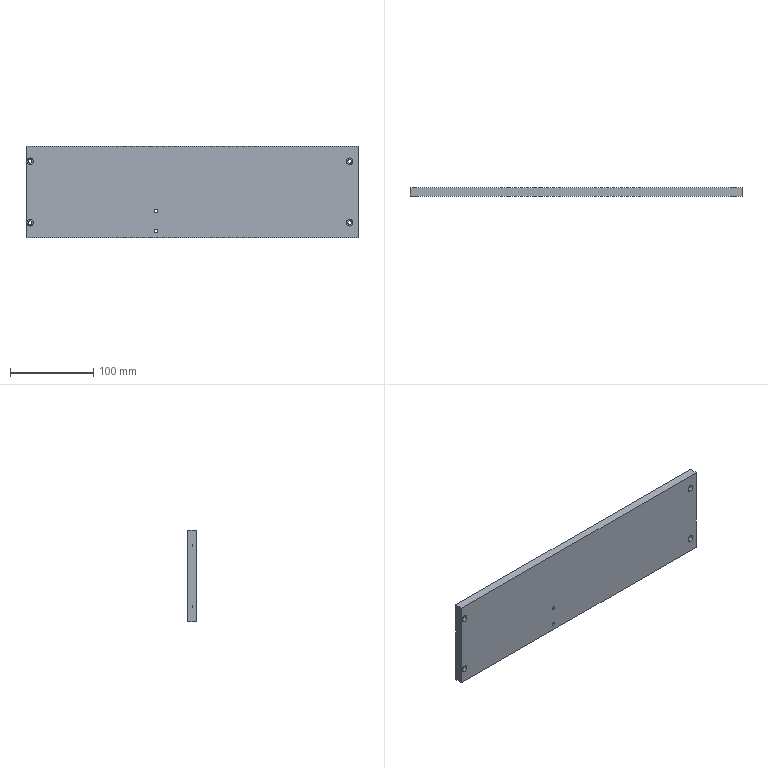Component | SolidWorks | CS021-A10-A001-1 | 1 solid | 30 faces | box 400 x 10 x 110 mm | volume 438454 mm3 | cylinder 20 | plane 10 | commonest cylinder face diameters 8 x8 4.5 x8 4.2 x4 | material AL6061
build123d program:
from build123d import *

# Parameters (mm, degrees)
SKETCH1_W                                          = 400
SKETCH1_H                                          = 110
BOSS_EXTRUDE1_DEPTH                                = 5
M5_TAPPED_HOLE1_D                                  = 4.2
HOLE_SIZE_ACCORDING_TO_SLOTTED_PAN_HEA_D           = 4.5
HOLE_SIZE_ACCORDING_TO_SLOTTED_PAN_HEA_CBORE_D     = 8
HOLE_SIZE_ACCORDING_TO_SLOTTED_PAN_HEA_CBORE_DEPTH = 4.6


with BuildPart() as part:
    # Sketch1 → Boss-Extrude1 (new, symmetric)
    with BuildSketch(Plane(origin=(0, 0, 0), x_dir=(1, 0, 0), z_dir=(0, 1, 0))):
        Rectangle(SKETCH1_W, SKETCH1_H)
    extrude(amount=BOSS_EXTRUDE1_DEPTH, both=True)

    # M5 Tapped Hole1 (through all)
    with Locations(Plane(origin=(0, 5, 0), x_dir=(1, 0, 0), z_dir=(0, 1, 0))):
        with Locations((-43.5, 47), (-43.5, 23)):
            Hole(M5_TAPPED_HOLE1_D / 2)

    # Hole Size _according to_ Slotted Pan Hea (through all)
    with Locations(Plane(origin=(0, -5, 0), x_dir=(-1, 0, 0), z_dir=(0, -1, 0))):
        with Locations((195, -37), (195, 37), (-190, -37), (-190, 37)):
            CounterBoreHole(HOLE_SIZE_ACCORDING_TO_SLOTTED_PAN_HEA_D / 2, HOLE_SIZE_ACCORDING_TO_SLOTTED_PAN_HEA_CBORE_D / 2, HOLE_SIZE_ACCORDING_TO_SLOTTED_PAN_HEA_CBORE_DEPTH)


solid = part.part

# Placed as in the assembly
solid = solid.moved(Location((35.949, 19.817, 0), (0, 0, 0)))
STEP:
#1=COLOUR_RGB('',0.7922,0.8196,0.9333);
#2=FILL_AREA_STYLE_COLOUR('',#1);
#3=FILL_AREA_STYLE('',(#2));
#4=SURFACE_STYLE_FILL_AREA(#3);
#5=SURFACE_SIDE_STYLE('',(#4));
#6=SURFACE_STYLE_USAGE(.BOTH.,#5);
#7=PRESENTATION_STYLE_ASSIGNMENT((#6));
#8=CARTESIAN_POINT('',(-6.262,0.7644,1.614));
#9=VERTEX_POINT('',#8);
#10=CARTESIAN_POINT('',(-6.262,0.7644,1.299));
#11=VERTEX_POINT('',#10);
#12=CARTESIAN_POINT('',(-6.262,0.7644,1.457));
#13=DIRECTION('',(0.,-1.,0.));
#14=DIRECTION('',(0.,0.,-1.));
#15=AXIS2_PLACEMENT_3D('',#12,#13,#14);
#16=CIRCLE('',#15,0.1575);
#17=EDGE_CURVE('',#9,#11,#16,.T.);
#18=ORIENTED_EDGE('',*,*,#17,.F.);
#19=CARTESIAN_POINT('',(-6.262,0.5833,1.614));
#20=VERTEX_POINT('',#19);
#21=CARTESIAN_POINT('',(-6.262,0.5833,1.614));
#22=DIRECTION('',(0.,-1.,0.));
#23=VECTOR('',#22,39.37);
#24=LINE('',#21,#23);
#25=EDGE_CURVE('',#9,#20,#24,.T.);
#26=ORIENTED_EDGE('',*,*,#25,.T.);
#27=CARTESIAN_POINT('',(-6.262,0.5833,1.299));
#28=VERTEX_POINT('',#27);
#29=CARTESIAN_POINT('',(-6.262,0.5833,1.457));
#30=DIRECTION('',(0.,-1.,0.));
#31=DIRECTION('',(0.,0.,-1.));
#32=AXIS2_PLACEMENT_3D('',#29,#30,#31);
#33=CIRCLE('',#32,0.1575);
#34=EDGE_CURVE('',#20,#28,#33,.T.);
#35=ORIENTED_EDGE('',*,*,#34,.T.);
#36=CARTESIAN_POINT('',(-6.262,0.5833,1.299));
#37=DIRECTION('',(0.,-1.,0.));
#38=VECTOR('',#37,39.37);
#39=LINE('',#36,#38);
#40=EDGE_CURVE('',#11,#28,#39,.T.);
#41=ORIENTED_EDGE('',*,*,#40,.F.);
#42=EDGE_LOOP('',(#18,#26,#35,#41));
#43=FACE_OUTER_BOUND('',#42,.T.);
#44=CARTESIAN_POINT('',(-6.262,0.5833,1.457));
#45=DIRECTION('',(0.,-1.,0.));
#46=DIRECTION('',(0.,0.,-1.));
#47=AXIS2_PLACEMENT_3D('',#44,#45,#46);
#48=CYLINDRICAL_SURFACE('',#47,0.1575);
#49=ADVANCED_FACE('',(#43),#48,.F.);
#50=CARTESIAN_POINT('',(-6.262,0.977,1.545));
#51=VERTEX_POINT('',#50);
#52=CARTESIAN_POINT('',(-6.262,0.977,1.368));
#53=VERTEX_POINT('',#52);
#54=CARTESIAN_POINT('',(-6.262,0.977,1.457));
#55=DIRECTION('',(0.,-1.,0.));
#56=DIRECTION('',(0.,0.,-1.));
#57=AXIS2_PLACEMENT_3D('',#54,#55,#56);
#58=CIRCLE('',#57,0.08858);
#59=EDGE_CURVE('',#51,#53,#58,.T.);
#60=ORIENTED_EDGE('',*,*,#59,.F.);
#61=CARTESIAN_POINT('',(-6.262,0.7644,1.545));
#62=VERTEX_POINT('',#61);
#63=CARTESIAN_POINT('',(-6.262,0.5833,1.545));
#64=DIRECTION('',(0.,-1.,0.));
#65=VECTOR('',#64,39.37);
#66=LINE('',#63,#65);
#67=EDGE_CURVE('',#51,#62,#66,.T.);
#68=ORIENTED_EDGE('',*,*,#67,.T.);
#69=CARTESIAN_POINT('',(-6.262,0.7644,1.368));
#70=VERTEX_POINT('',#69);
#71=CARTESIAN_POINT('',(-6.262,0.7644,1.457));
#72=DIRECTION('',(0.,-1.,0.));
#73=DIRECTION('',(0.,0.,-1.));
#74=AXIS2_PLACEMENT_3D('',#71,#72,#73);
#75=CIRCLE('',#74,0.08858);
#76=EDGE_CURVE('',#62,#70,#75,.T.);
#77=ORIENTED_EDGE('',*,*,#76,.T.);
#78=CARTESIAN_POINT('',(-6.262,0.5833,1.368));
#79=DIRECTION('',(0.,-1.,0.));
#80=VECTOR('',#79,39.37);
#81=LINE('',#78,#80);
#82=EDGE_CURVE('',#53,#70,#81,.T.);
#83=ORIENTED_EDGE('',*,*,#82,.F.);
#84=EDGE_LOOP('',(#60,#68,#77,#83));
#85=FACE_OUTER_BOUND('',#84,.T.);
#86=CARTESIAN_POINT('',(-6.262,0.5833,1.457));
#87=DIRECTION('',(0.,-1.,0.));
#88=DIRECTION('',(0.,0.,-1.));
#89=AXIS2_PLACEMENT_3D('',#86,#87,#88);
#90=CYLINDRICAL_SURFACE('',#89,0.08858);
#91=ADVANCED_FACE('',(#85),#90,.F.);
#92=CARTESIAN_POINT('',(-6.262,0.7644,-1.299));
#93=VERTEX_POINT('',#92);
#94=CARTESIAN_POINT('',(-6.262,0.7644,-1.614));
#95=VERTEX_POINT('',#94);
#96=CARTESIAN_POINT('',(-6.262,0.7644,-1.457));
#97=DIRECTION('',(0.,-1.,0.));
#98=DIRECTION('',(0.,0.,-1.));
#99=AXIS2_PLACEMENT_3D('',#96,#97,#98);
#100=CIRCLE('',#99,0.1575);
#101=EDGE_CURVE('',#93,#95,#100,.T.);
#102=ORIENTED_EDGE('',*,*,#101,.F.);
#103=CARTESIAN_POINT('',(-6.262,0.5833,-1.299));
#104=VERTEX_POINT('',#103);
#105=CARTESIAN_POINT('',(-6.262,0.5833,-1.299));
#106=DIRECTION('',(0.,-1.,0.));
#107=VECTOR('',#106,39.37);
#108=LINE('',#105,#107);
#109=EDGE_CURVE('',#93,#104,#108,.T.);
#110=ORIENTED_EDGE('',*,*,#109,.T.);
#111=CARTESIAN_POINT('',(-6.262,0.5833,-1.614));
#112=VERTEX_POINT('',#111);
#113=CARTESIAN_POINT('',(-6.262,0.5833,-1.457));
#114=DIRECTION('',(0.,-1.,0.));
#115=DIRECTION('',(0.,0.,-1.));
#116=AXIS2_PLACEMENT_3D('',#113,#114,#115);
#117=CIRCLE('',#116,0.1575);
#118=EDGE_CURVE('',#104,#112,#117,.T.);
#119=ORIENTED_EDGE('',*,*,#118,.T.);
#120=CARTESIAN_POINT('',(-6.262,0.5833,-1.614));
#121=DIRECTION('',(0.,-1.,0.));
#122=VECTOR('',#121,39.37);
#123=LINE('',#120,#122);
#124=EDGE_CURVE('',#95,#112,#123,.T.);
#125=ORIENTED_EDGE('',*,*,#124,.F.);
#126=EDGE_LOOP('',(#102,#110,#119,#125));
#127=FACE_OUTER_BOUND('',#126,.T.);
#128=CARTESIAN_POINT('',(-6.262,0.5833,-1.457));
#129=DIRECTION('',(0.,-1.,0.));
#130=DIRECTION('',(0.,0.,-1.));
#131=AXIS2_PLACEMENT_3D('',#128,#129,#130);
#132=CYLINDRICAL_SURFACE('',#131,0.1575);
#133=ADVANCED_FACE('',(#127),#132,.F.);
#134=CARTESIAN_POINT('',(-6.262,0.977,-1.368));
#135=VERTEX_POINT('',#134);
#136=CARTESIAN_POINT('',(-6.262,0.977,-1.545));
#137=VERTEX_POINT('',#136);
#138=CARTESIAN_POINT('',(-6.262,0.977,-1.457));
#139=DIRECTION('',(0.,-1.,0.));
#140=DIRECTION('',(0.,0.,-1.));
#141=AXIS2_PLACEMENT_3D('',#138,#139,#140);
#142=CIRCLE('',#141,0.08858);
#143=EDGE_CURVE('',#135,#137,#142,.T.);
#144=ORIENTED_EDGE('',*,*,#143,.F.);
#145=CARTESIAN_POINT('',(-6.262,0.7644,-1.368));
#146=VERTEX_POINT('',#145);
#147=CARTESIAN_POINT('',(-6.262,0.5833,-1.368));
#148=DIRECTION('',(0.,-1.,0.));
#149=VECTOR('',#148,39.37);
#150=LINE('',#147,#149);
#151=EDGE_CURVE('',#135,#146,#150,.T.);
#152=ORIENTED_EDGE('',*,*,#151,.T.);
#153=CARTESIAN_POINT('',(-6.262,0.7644,-1.545));
#154=VERTEX_POINT('',#153);
#155=CARTESIAN_POINT('',(-6.262,0.7644,-1.457));
#156=DIRECTION('',(0.,-1.,0.));
#157=DIRECTION('',(0.,0.,-1.));
#158=AXIS2_PLACEMENT_3D('',#155,#156,#157);
#159=CIRCLE('',#158,0.08858);
#160=EDGE_CURVE('',#146,#154,#159,.T.);
#161=ORIENTED_EDGE('',*,*,#160,.T.);
#162=CARTESIAN_POINT('',(-6.262,0.5833,-1.545));
#163=DIRECTION('',(0.,-1.,0.));
#164=VECTOR('',#163,39.37);
#165=LINE('',#162,#164);
#166=EDGE_CURVE('',#137,#154,#165,.T.);
#167=ORIENTED_EDGE('',*,*,#166,.F.);
#168=EDGE_LOOP('',(#144,#152,#161,#167));
#169=FACE_OUTER_BOUND('',#168,.T.);
#170=CARTESIAN_POINT('',(-6.262,0.5833,-1.457));
#171=DIRECTION('',(0.,-1.,0.));
#172=DIRECTION('',(0.,0.,-1.));
#173=AXIS2_PLACEMENT_3D('',#170,#171,#172);
#174=CYLINDRICAL_SURFACE('',#173,0.08858);
#175=ADVANCED_FACE('',(#169),#174,.F.);
#176=CARTESIAN_POINT('',(8.896,0.7644,1.614));
#177=VERTEX_POINT('',#176);
#178=CARTESIAN_POINT('',(8.896,0.7644,1.299));
#179=VERTEX_POINT('',#178);
#180=CARTESIAN_POINT('',(8.896,0.7644,1.457));
#181=DIRECTION('',(0.,-1.,0.));
#182=DIRECTION('',(0.,0.,-1.));
#183=AXIS2_PLACEMENT_3D('',#180,#181,#182);
#184=CIRCLE('',#183,0.1575);
#185=EDGE_CURVE('',#177,#179,#184,.T.);
#186=ORIENTED_EDGE('',*,*,#185,.F.);
#187=CARTESIAN_POINT('',(8.896,0.5833,1.614));
#188=VERTEX_POINT('',#187);
#189=CARTESIAN_POINT('',(8.896,0.5833,1.614));
#190=DIRECTION('',(0.,-1.,0.));
#191=VECTOR('',#190,39.37);
#192=LINE('',#189,#191);
#193=EDGE_CURVE('',#177,#188,#192,.T.);
#194=ORIENTED_EDGE('',*,*,#193,.T.);
#195=CARTESIAN_POINT('',(8.896,0.5833,1.299));
#196=VERTEX_POINT('',#195);
#197=CARTESIAN_POINT('',(8.896,0.5833,1.457));
#198=DIRECTION('',(0.,-1.,0.));
#199=DIRECTION('',(0.,0.,-1.));
#200=AXIS2_PLACEMENT_3D('',#197,#198,#199);
#201=CIRCLE('',#200,0.1575);
#202=EDGE_CURVE('',#188,#196,#201,.T.);
#203=ORIENTED_EDGE('',*,*,#202,.T.);
#204=CARTESIAN_POINT('',(8.896,0.5833,1.299));
#205=DIRECTION('',(0.,-1.,0.));
#206=VECTOR('',#205,39.37);
#207=LINE('',#204,#206);
#208=EDGE_CURVE('',#179,#196,#207,.T.);
#209=ORIENTED_EDGE('',*,*,#208,.F.);
#210=EDGE_LOOP('',(#186,#194,#203,#209));
#211=FACE_OUTER_BOUND('',#210,.T.);
#212=CARTESIAN_POINT('',(8.896,0.5833,1.457));
#213=DIRECTION('',(0.,-1.,0.));
#214=DIRECTION('',(0.,0.,-1.));
#215=AXIS2_PLACEMENT_3D('',#212,#213,#214);
#216=CYLINDRICAL_SURFACE('',#215,0.1575);
#217=ADVANCED_FACE('',(#211),#216,.F.);
#218=CARTESIAN_POINT('',(8.896,0.977,1.545));
#219=VERTEX_POINT('',#218);
#220=CARTESIAN_POINT('',(8.896,0.977,1.368));
#221=VERTEX_POINT('',#220);
#222=CARTESIAN_POINT('',(8.896,0.977,1.457));
#223=DIRECTION('',(0.,-1.,0.));
#224=DIRECTION('',(0.,0.,-1.));
#225=AXIS2_PLACEMENT_3D('',#222,#223,#224);
#226=CIRCLE('',#225,0.08858);
#227=EDGE_CURVE('',#219,#221,#226,.T.);
#228=ORIENTED_EDGE('',*,*,#227,.F.);
#229=CARTESIAN_POINT('',(8.896,0.7644,1.545));
#230=VERTEX_POINT('',#229);
#231=CARTESIAN_POINT('',(8.896,0.5833,1.545));
#232=DIRECTION('',(0.,-1.,0.));
#233=VECTOR('',#232,39.37);
#234=LINE('',#231,#233);
#235=EDGE_CURVE('',#219,#230,#234,.T.);
#236=ORIENTED_EDGE('',*,*,#235,.T.);
#237=CARTESIAN_POINT('',(8.896,0.7644,1.368));
#238=VERTEX_POINT('',#237);
#239=CARTESIAN_POINT('',(8.896,0.7644,1.457));
#240=DIRECTION('',(0.,-1.,0.));
#241=DIRECTION('',(0.,0.,-1.));
#242=AXIS2_PLACEMENT_3D('',#239,#240,#241);
#243=CIRCLE('',#242,0.08858);
#244=EDGE_CURVE('',#230,#238,#243,.T.);
#245=ORIENTED_EDGE('',*,*,#244,.T.);
#246=CARTESIAN_POINT('',(8.896,0.5833,1.368));
#247=DIRECTION('',(0.,-1.,0.));
#248=VECTOR('',#247,39.37);
#249=LINE('',#246,#248);
#250=EDGE_CURVE('',#221,#238,#249,.T.);
#251=ORIENTED_EDGE('',*,*,#250,.F.);
#252=EDGE_LOOP('',(#228,#236,#245,#251));
#253=FACE_OUTER_BOUND('',#252,.T.);
#254=CARTESIAN_POINT('',(8.896,0.5833,1.457));
#255=DIRECTION('',(0.,-1.,0.));
#256=DIRECTION('',(0.,0.,-1.));
#257=AXIS2_PLACEMENT_3D('',#254,#255,#256);
#258=CYLINDRICAL_SURFACE('',#257,0.08858);
#259=ADVANCED_FACE('',(#253),#258,.F.);
#260=CARTESIAN_POINT('',(8.896,0.7644,-1.299));
#261=VERTEX_POINT('',#260);
#262=CARTESIAN_POINT('',(8.896,0.7644,-1.614));
#263=VERTEX_POINT('',#262);
#264=CARTESIAN_POINT('',(8.896,0.7644,-1.457));
#265=DIRECTION('',(0.,-1.,0.));
#266=DIRECTION('',(0.,0.,-1.));
#267=AXIS2_PLACEMENT_3D('',#264,#265,#266);
#268=CIRCLE('',#267,0.1575);
#269=EDGE_CURVE('',#261,#263,#268,.T.);
#270=ORIENTED_EDGE('',*,*,#269,.F.);
#271=CARTESIAN_POINT('',(8.896,0.5833,-1.299));
#272=VERTEX_POINT('',#271);
#273=CARTESIAN_POINT('',(8.896,0.5833,-1.299));
#274=DIRECTION('',(0.,-1.,0.));
#275=VECTOR('',#274,39.37);
#276=LINE('',#273,#275);
#277=EDGE_CURVE('',#261,#272,#276,.T.);
#278=ORIENTED_EDGE('',*,*,#277,.T.);
#279=CARTESIAN_POINT('',(8.896,0.5833,-1.614));
#280=VERTEX_POINT('',#279);
#281=CARTESIAN_POINT('',(8.896,0.5833,-1.457));
#282=DIRECTION('',(0.,-1.,0.));
#283=DIRECTION('',(0.,0.,-1.));
#284=AXIS2_PLACEMENT_3D('',#281,#282,#283);
#285=CIRCLE('',#284,0.1575);
#286=EDGE_CURVE('',#272,#280,#285,.T.);
#287=ORIENTED_EDGE('',*,*,#286,.T.);
#288=CARTESIAN_POINT('',(8.896,0.5833,-1.614));
#289=DIRECTION('',(0.,-1.,0.));
#290=VECTOR('',#289,39.37);
#291=LINE('',#288,#290);
#292=EDGE_CURVE('',#263,#280,#291,.T.);
#293=ORIENTED_EDGE('',*,*,#292,.F.);
#294=EDGE_LOOP('',(#270,#278,#287,#293));
#295=FACE_OUTER_BOUND('',#294,.T.);
#296=CARTESIAN_POINT('',(8.896,0.5833,-1.457));
#297=DIRECTION('',(0.,-1.,0.));
#298=DIRECTION('',(0.,0.,-1.));
#299=AXIS2_PLACEMENT_3D('',#296,#297,#298);
#300=CYLINDRICAL_SURFACE('',#299,0.1575);
#301=ADVANCED_FACE('',(#295),#300,.F.);
#302=CARTESIAN_POINT('',(8.896,0.977,-1.368));
#303=VERTEX_POINT('',#302);
#304=CARTESIAN_POINT('',(8.896,0.977,-1.545));
#305=VERTEX_POINT('',#304);
#306=CARTESIAN_POINT('',(8.896,0.977,-1.457));
#307=DIRECTION('',(0.,-1.,0.));
#308=DIRECTION('',(0.,0.,-1.));
#309=AXIS2_PLACEMENT_3D('',#306,#307,#308);
#310=CIRCLE('',#309,0.08858);
#311=EDGE_CURVE('',#303,#305,#310,.T.);
#312=ORIENTED_EDGE('',*,*,#311,.F.);
#313=CARTESIAN_POINT('',(8.896,0.7644,-1.368));
#314=VERTEX_POINT('',#313);
#315=CARTESIAN_POINT('',(8.896,0.5833,-1.368));
#316=DIRECTION('',(0.,-1.,0.));
#317=VECTOR('',#316,39.37);
#318=LINE('',#315,#317);
#319=EDGE_CURVE('',#303,#314,#318,.T.);
#320=ORIENTED_EDGE('',*,*,#319,.T.);
#321=CARTESIAN_POINT('',(8.896,0.7644,-1.545));
#322=VERTEX_POINT('',#321);
#323=CARTESIAN_POINT('',(8.896,0.7644,-1.457));
#324=DIRECTION('',(0.,-1.,0.));
#325=DIRECTION('',(0.,0.,-1.));
#326=AXIS2_PLACEMENT_3D('',#323,#324,#325);
#327=CIRCLE('',#326,0.08858);
#328=EDGE_CURVE('',#314,#322,#327,.T.);
#329=ORIENTED_EDGE('',*,*,#328,.T.);
#330=CARTESIAN_POINT('',(8.896,0.5833,-1.545));
#331=DIRECTION('',(0.,-1.,0.));
#332=VECTOR('',#331,39.37);
#333=LINE('',#330,#332);
#334=EDGE_CURVE('',#305,#322,#333,.T.);
#335=ORIENTED_EDGE('',*,*,#334,.F.);
#336=EDGE_LOOP('',(#312,#320,#329,#335));
#337=FACE_OUTER_BOUND('',#336,.T.);
#338=CARTESIAN_POINT('',(8.896,0.5833,-1.457));
#339=DIRECTION('',(0.,-1.,0.));
#340=DIRECTION('',(0.,0.,-1.));
#341=AXIS2_PLACEMENT_3D('',#338,#339,#340);
#342=CYLINDRICAL_SURFACE('',#341,0.08858);
#343=ADVANCED_FACE('',(#337),#342,.F.);
#344=CARTESIAN_POINT('',(-0.2973,0.5833,-1.933));
#345=VERTEX_POINT('',#344);
#346=CARTESIAN_POINT('',(-0.2973,0.5833,-1.768));
#347=VERTEX_POINT('',#346);
#348=CARTESIAN_POINT('',(-0.2973,0.5833,-1.85));
#349=DIRECTION('',(0.,1.,0.));
#350=DIRECTION('',(0.,0.,1.));
#351=AXIS2_PLACEMENT_3D('',#348,#349,#350);
#352=CIRCLE('',#351,0.08268);
#353=EDGE_CURVE('',#345,#347,#352,.T.);
#354=ORIENTED_EDGE('',*,*,#353,.F.);
#355=CARTESIAN_POINT('',(-0.2973,0.977,-1.933));
#356=VERTEX_POINT('',#355);
#357=CARTESIAN_POINT('',(-0.2973,0.977,-1.933));
#358=DIRECTION('',(0.,1.,0.));
#359=VECTOR('',#358,39.37);
#360=LINE('',#357,#359);
#361=EDGE_CURVE('',#345,#356,#360,.T.);
#362=ORIENTED_EDGE('',*,*,#361,.T.);
#363=CARTESIAN_POINT('',(-0.2973,0.977,-1.768));
#364=VERTEX_POINT('',#363);
#365=CARTESIAN_POINT('',(-0.2973,0.977,-1.85));
#366=DIRECTION('',(0.,1.,0.));
#367=DIRECTION('',(0.,0.,1.));
#368=AXIS2_PLACEMENT_3D('',#365,#366,#367);
#369=CIRCLE('',#368,0.08268);
#370=EDGE_CURVE('',#356,#364,#369,.T.);
#371=ORIENTED_EDGE('',*,*,#370,.T.);
#372=CARTESIAN_POINT('',(-0.2973,0.977,-1.768));
#373=DIRECTION('',(0.,1.,0.));
#374=VECTOR('',#373,39.37);
#375=LINE('',#372,#374);
#376=EDGE_CURVE('',#347,#364,#375,.T.);
#377=ORIENTED_EDGE('',*,*,#376,.F.);
#378=EDGE_LOOP('',(#354,#362,#371,#377));
#379=FACE_OUTER_BOUND('',#378,.T.);
#380=CARTESIAN_POINT('',(-0.2973,0.977,-1.85));
#381=DIRECTION('',(0.,1.,0.));
#382=DIRECTION('',(0.,0.,1.));
#383=AXIS2_PLACEMENT_3D('',#380,#381,#382);
#384=CYLINDRICAL_SURFACE('',#383,0.08268);
#385=ADVANCED_FACE('',(#379),#384,.F.);
#386=CARTESIAN_POINT('',(-0.2973,0.5833,-0.9882));
#387=VERTEX_POINT('',#386);
#388=CARTESIAN_POINT('',(-0.2973,0.5833,-0.8228));
#389=VERTEX_POINT('',#388);
#390=CARTESIAN_POINT('',(-0.2973,0.5833,-0.9055));
#391=DIRECTION('',(0.,1.,0.));
#392=DIRECTION('',(0.,0.,1.));
#393=AXIS2_PLACEMENT_3D('',#390,#391,#392);
#394=CIRCLE('',#393,0.08268);
#395=EDGE_CURVE('',#387,#389,#394,.T.);
#396=ORIENTED_EDGE('',*,*,#395,.F.);
#397=CARTESIAN_POINT('',(-0.2973,0.977,-0.9882));
#398=VERTEX_POINT('',#397);
#399=CARTESIAN_POINT('',(-0.2973,0.977,-0.9882));
#400=DIRECTION('',(0.,1.,0.));
#401=VECTOR('',#400,39.37);
#402=LINE('',#399,#401);
#403=EDGE_CURVE('',#387,#398,#402,.T.);
#404=ORIENTED_EDGE('',*,*,#403,.T.);
#405=CARTESIAN_POINT('',(-0.2973,0.977,-0.8228));
#406=VERTEX_POINT('',#405);
#407=CARTESIAN_POINT('',(-0.2973,0.977,-0.9055));
#408=DIRECTION('',(0.,1.,0.));
#409=DIRECTION('',(0.,0.,1.));
#410=AXIS2_PLACEMENT_3D('',#407,#408,#409);
#411=CIRCLE('',#410,0.08268);
#412=EDGE_CURVE('',#398,#406,#411,.T.);
#413=ORIENTED_EDGE('',*,*,#412,.T.);
#414=CARTESIAN_POINT('',(-0.2973,0.977,-0.8228));
#415=DIRECTION('',(0.,1.,0.));
#416=VECTOR('',#415,39.37);
#417=LINE('',#414,#416);
#418=EDGE_CURVE('',#389,#406,#417,.T.);
#419=ORIENTED_EDGE('',*,*,#418,.F.);
#420=EDGE_LOOP('',(#396,#404,#413,#419));
#421=FACE_OUTER_BOUND('',#420,.T.);
#422=CARTESIAN_POINT('',(-0.2973,0.977,-0.9055));
#423=DIRECTION('',(0.,1.,0.));
#424=DIRECTION('',(0.,0.,1.));
#425=AXIS2_PLACEMENT_3D('',#422,#423,#424);
#426=CYLINDRICAL_SURFACE('',#425,0.08268);
#427=ADVANCED_FACE('',(#421),#426,.F.);
#428=CARTESIAN_POINT('',(9.289,0.5833,2.165));
#429=VERTEX_POINT('',#428);
#430=CARTESIAN_POINT('',(9.289,0.5833,-2.165));
#431=VERTEX_POINT('',#430);
#432=CARTESIAN_POINT('',(9.289,0.5833,2.165));
#433=DIRECTION('',(0.,0.,-1.));
#434=VECTOR('',#433,39.37);
#435=LINE('',#432,#434);
#436=EDGE_CURVE('',#429,#431,#435,.T.);
#437=ORIENTED_EDGE('',*,*,#436,.T.);
#438=CARTESIAN_POINT('',(9.289,0.977,-2.165));
#439=VERTEX_POINT('',#438);
#440=CARTESIAN_POINT('',(9.289,0.977,-2.165));
#441=DIRECTION('',(0.,-1.,0.));
#442=VECTOR('',#441,39.37);
#443=LINE('',#440,#442);
#444=EDGE_CURVE('',#439,#431,#443,.T.);
#445=ORIENTED_EDGE('',*,*,#444,.F.);
#446=CARTESIAN_POINT('',(9.289,0.977,2.165));
#447=VERTEX_POINT('',#446);
#448=CARTESIAN_POINT('',(9.289,0.977,2.165));
#449=DIRECTION('',(0.,0.,-1.));
#450=VECTOR('',#449,39.37);
#451=LINE('',#448,#450);
#452=EDGE_CURVE('',#447,#439,#451,.T.);
#453=ORIENTED_EDGE('',*,*,#452,.F.);
#454=CARTESIAN_POINT('',(9.289,0.977,2.165));
#455=DIRECTION('',(0.,-1.,0.));
#456=VECTOR('',#455,39.37);
#457=LINE('',#454,#456);
#458=EDGE_CURVE('',#447,#429,#457,.T.);
#459=ORIENTED_EDGE('',*,*,#458,.T.);
#460=EDGE_LOOP('',(#437,#445,#453,#459));
#461=FACE_OUTER_BOUND('',#460,.T.);
#462=CARTESIAN_POINT('',(9.289,0.977,2.165));
#463=DIRECTION('',(-1.,0.,0.));
#464=DIRECTION('',(0.,0.,1.));
#465=AXIS2_PLACEMENT_3D('',#462,#463,#464);
#466=PLANE('',#465);
#467=ADVANCED_FACE('',(#461),#466,.F.);
#468=CARTESIAN_POINT('',(-6.459,0.5833,-2.165));
#469=VERTEX_POINT('',#468);
#470=CARTESIAN_POINT('',(-6.459,0.5833,-2.165));
#471=DIRECTION('',(-1.,0.,0.));
#472=VECTOR('',#471,39.37);
#473=LINE('',#470,#472);
#474=EDGE_CURVE('',#431,#469,#473,.T.);
#475=ORIENTED_EDGE('',*,*,#474,.T.);
#476=CARTESIAN_POINT('',(-6.459,0.977,-2.165));
#477=VERTEX_POINT('',#476);
#478=CARTESIAN_POINT('',(-6.459,0.977,-2.165));
#479=DIRECTION('',(0.,-1.,0.));
#480=VECTOR('',#479,39.37);
#481=LINE('',#478,#480);
#482=EDGE_CURVE('',#477,#469,#481,.T.);
#483=ORIENTED_EDGE('',*,*,#482,.F.);
#484=CARTESIAN_POINT('',(-6.459,0.977,-2.165));
#485=DIRECTION('',(-1.,0.,0.));
#486=VECTOR('',#485,39.37);
#487=LINE('',#484,#486);
#488=EDGE_CURVE('',#439,#477,#487,.T.);
#489=ORIENTED_EDGE('',*,*,#488,.F.);
#490=ORIENTED_EDGE('',*,*,#444,.T.);
#491=EDGE_LOOP('',(#475,#483,#489,#490));
#492=FACE_OUTER_BOUND('',#491,.T.);
#493=CARTESIAN_POINT('',(-6.459,0.977,-2.165));
#494=DIRECTION('',(0.,0.,1.));
#495=DIRECTION('',(1.,0.,0.));
#496=AXIS2_PLACEMENT_3D('',#493,#494,#495);
#497=PLANE('',#496);
#498=ADVANCED_FACE('',(#492),#497,.F.);
#499=CARTESIAN_POINT('',(-6.459,0.5833,2.165));
#500=VERTEX_POINT('',#499);
#501=CARTESIAN_POINT('',(-6.459,0.5833,2.165));
#502=DIRECTION('',(0.,0.,1.));
#503=VECTOR('',#502,39.37);
#504=LINE('',#501,#503);
#505=EDGE_CURVE('',#469,#500,#504,.T.);
#506=ORIENTED_EDGE('',*,*,#505,.T.);
#507=CARTESIAN_POINT('',(-6.459,0.977,2.165));
#508=VERTEX_POINT('',#507);
#509=CARTESIAN_POINT('',(-6.459,0.977,2.165));
#510=DIRECTION('',(0.,-1.,0.));
#511=VECTOR('',#510,39.37);
#512=LINE('',#509,#511);
#513=EDGE_CURVE('',#508,#500,#512,.T.);
#514=ORIENTED_EDGE('',*,*,#513,.F.);
#515=CARTESIAN_POINT('',(-6.459,0.977,2.165));
#516=DIRECTION('',(0.,0.,1.));
#517=VECTOR('',#516,39.37);
#518=LINE('',#515,#517);
#519=EDGE_CURVE('',#477,#508,#518,.T.);
#520=ORIENTED_EDGE('',*,*,#519,.F.);
#521=ORIENTED_EDGE('',*,*,#482,.T.);
#522=EDGE_LOOP('',(#506,#514,#520,#521));
#523=FACE_OUTER_BOUND('',#522,.T.);
#524=CARTESIAN_POINT('',(-6.459,0.977,2.165));
#525=DIRECTION('',(1.,0.,0.));
#526=DIRECTION('',(0.,0.,-1.));
#527=AXIS2_PLACEMENT_3D('',#524,#525,#526);
#528=PLANE('',#527);
#529=ADVANCED_FACE('',(#523),#528,.F.);
#530=CARTESIAN_POINT('',(-6.459,0.5833,2.165));
#531=DIRECTION('',(1.,0.,0.));
#532=VECTOR('',#531,39.37);
#533=LINE('',#530,#532);
#534=EDGE_CURVE('',#500,#429,#533,.T.);
#535=ORIENTED_EDGE('',*,*,#534,.T.);
#536=ORIENTED_EDGE('',*,*,#458,.F.);
#537=CARTESIAN_POINT('',(-6.459,0.977,2.165));
#538=DIRECTION('',(1.,0.,0.));
#539=VECTOR('',#538,39.37);
#540=LINE('',#537,#539);
#541=EDGE_CURVE('',#508,#447,#540,.T.);
#542=ORIENTED_EDGE('',*,*,#541,.F.);
#543=ORIENTED_EDGE('',*,*,#513,.T.);
#544=EDGE_LOOP('',(#535,#536,#542,#543));
#545=FACE_OUTER_BOUND('',#544,.T.);
#546=CARTESIAN_POINT('',(-6.459,0.977,2.165));
#547=DIRECTION('',(0.,0.,-1.));
#548=DIRECTION('',(-1.,0.,0.));
#549=AXIS2_PLACEMENT_3D('',#546,#547,#548);
#550=PLANE('',#549);
#551=ADVANCED_FACE('',(#545),#550,.F.);
#552=CARTESIAN_POINT('',(-6.262,0.977,1.457));
#553=DIRECTION('',(0.,-1.,0.));
#554=DIRECTION('',(0.,0.,-1.));
#555=AXIS2_PLACEMENT_3D('',#552,#553,#554);
#556=CIRCLE('',#555,0.08858);
#557=EDGE_CURVE('',#53,#51,#556,.T.);
#558=ORIENTED_EDGE('',*,*,#557,.T.);
#559=ORIENTED_EDGE('',*,*,#59,.T.);
#560=EDGE_LOOP('',(#558,#559));
#561=FACE_BOUND('',#560,.T.);
#562=CARTESIAN_POINT('',(-6.262,0.977,-1.457));
#563=DIRECTION('',(0.,-1.,0.));
#564=DIRECTION('',(0.,0.,-1.));
#565=AXIS2_PLACEMENT_3D('',#562,#563,#564);
#566=CIRCLE('',#565,0.08858);
#567=EDGE_CURVE('',#137,#135,#566,.T.);
#568=ORIENTED_EDGE('',*,*,#567,.T.);
#569=ORIENTED_EDGE('',*,*,#143,.T.);
#570=EDGE_LOOP('',(#568,#569));
#571=FACE_BOUND('',#570,.T.);
#572=CARTESIAN_POINT('',(8.896,0.977,1.457));
#573=DIRECTION('',(0.,-1.,0.));
#574=DIRECTION('',(0.,0.,-1.));
#575=AXIS2_PLACEMENT_3D('',#572,#573,#574);
#576=CIRCLE('',#575,0.08858);
#577=EDGE_CURVE('',#221,#219,#576,.T.);
#578=ORIENTED_EDGE('',*,*,#577,.T.);
#579=ORIENTED_EDGE('',*,*,#227,.T.);
#580=EDGE_LOOP('',(#578,#579));
#581=FACE_BOUND('',#580,.T.);
#582=CARTESIAN_POINT('',(8.896,0.977,-1.457));
#583=DIRECTION('',(0.,-1.,0.));
#584=DIRECTION('',(0.,0.,-1.));
#585=AXIS2_PLACEMENT_3D('',#582,#583,#584);
#586=CIRCLE('',#585,0.08858);
#587=EDGE_CURVE('',#305,#303,#586,.T.);
#588=ORIENTED_EDGE('',*,*,#587,.T.);
#589=ORIENTED_EDGE('',*,*,#311,.T.);
#590=EDGE_LOOP('',(#588,#589));
#591=FACE_BOUND('',#590,.T.);
#592=CARTESIAN_POINT('',(-0.2973,0.977,-1.85));
#593=DIRECTION('',(0.,1.,0.));
#594=DIRECTION('',(0.,0.,1.));
#595=AXIS2_PLACEMENT_3D('',#592,#593,#594);
#596=CIRCLE('',#595,0.08268);
#597=EDGE_CURVE('',#364,#356,#596,.T.);
#598=ORIENTED_EDGE('',*,*,#597,.F.);
#599=ORIENTED_EDGE('',*,*,#370,.F.);
#600=EDGE_LOOP('',(#598,#599));
#601=FACE_BOUND('',#600,.T.);
#602=CARTESIAN_POINT('',(-0.2973,0.977,-0.9055));
#603=DIRECTION('',(0.,1.,0.));
#604=DIRECTION('',(0.,0.,1.));
#605=AXIS2_PLACEMENT_3D('',#602,#603,#604);
#606=CIRCLE('',#605,0.08268);
#607=EDGE_CURVE('',#406,#398,#606,.T.);
#608=ORIENTED_EDGE('',*,*,#607,.F.);
#609=ORIENTED_EDGE('',*,*,#412,.F.);
#610=EDGE_LOOP('',(#608,#609));
#611=FACE_BOUND('',#610,.T.);
#612=ORIENTED_EDGE('',*,*,#452,.T.);
#613=ORIENTED_EDGE('',*,*,#488,.T.);
#614=ORIENTED_EDGE('',*,*,#519,.T.);
#615=ORIENTED_EDGE('',*,*,#541,.T.);
#616=EDGE_LOOP('',(#612,#613,#614,#615));
#617=FACE_OUTER_BOUND('',#616,.T.);
#618=CARTESIAN_POINT('',(1.415,0.977,0.));
#619=DIRECTION('',(0.,-1.,0.));
#620=DIRECTION('',(0.,0.,-1.));
#621=AXIS2_PLACEMENT_3D('',#618,#619,#620);
#622=PLANE('',#621);
#623=ADVANCED_FACE('',(#561,#571,#581,#591,#601,#611,#617),#622,.F.);
#624=CARTESIAN_POINT('',(-6.262,0.5833,1.457));
#625=DIRECTION('',(0.,-1.,0.));
#626=DIRECTION('',(0.,0.,-1.));
#627=AXIS2_PLACEMENT_3D('',#624,#625,#626);
#628=CIRCLE('',#627,0.1575);
#629=EDGE_CURVE('',#28,#20,#628,.T.);
#630=ORIENTED_EDGE('',*,*,#629,.F.);
#631=ORIENTED_EDGE('',*,*,#34,.F.);
#632=EDGE_LOOP('',(#630,#631));
#633=FACE_BOUND('',#632,.T.);
#634=CARTESIAN_POINT('',(-6.262,0.5833,-1.457));
#635=DIRECTION('',(0.,-1.,0.));
#636=DIRECTION('',(0.,0.,-1.));
#637=AXIS2_PLACEMENT_3D('',#634,#635,#636);
#638=CIRCLE('',#637,0.1575);
#639=EDGE_CURVE('',#112,#104,#638,.T.);
#640=ORIENTED_EDGE('',*,*,#639,.F.);
#641=ORIENTED_EDGE('',*,*,#118,.F.);
#642=EDGE_LOOP('',(#640,#641));
#643=FACE_BOUND('',#642,.T.);
#644=CARTESIAN_POINT('',(8.896,0.5833,1.457));
#645=DIRECTION('',(0.,-1.,0.));
#646=DIRECTION('',(0.,0.,-1.));
#647=AXIS2_PLACEMENT_3D('',#644,#645,#646);
#648=CIRCLE('',#647,0.1575);
#649=EDGE_CURVE('',#196,#188,#648,.T.);
#650=ORIENTED_EDGE('',*,*,#649,.F.);
#651=ORIENTED_EDGE('',*,*,#202,.F.);
#652=EDGE_LOOP('',(#650,#651));
#653=FACE_BOUND('',#652,.T.);
#654=CARTESIAN_POINT('',(8.896,0.5833,-1.457));
#655=DIRECTION('',(0.,-1.,0.));
#656=DIRECTION('',(0.,0.,-1.));
#657=AXIS2_PLACEMENT_3D('',#654,#655,#656);
#658=CIRCLE('',#657,0.1575);
#659=EDGE_CURVE('',#280,#272,#658,.T.);
#660=ORIENTED_EDGE('',*,*,#659,.F.);
#661=ORIENTED_EDGE('',*,*,#286,.F.);
#662=EDGE_LOOP('',(#660,#661));
#663=FACE_BOUND('',#662,.T.);
#664=CARTESIAN_POINT('',(-0.2973,0.5833,-1.85));
#665=DIRECTION('',(0.,1.,0.));
#666=DIRECTION('',(0.,0.,1.));
#667=AXIS2_PLACEMENT_3D('',#664,#665,#666);
#668=CIRCLE('',#667,0.08268);
#669=EDGE_CURVE('',#347,#345,#668,.T.);
#670=ORIENTED_EDGE('',*,*,#669,.T.);
#671=ORIENTED_EDGE('',*,*,#353,.T.);
#672=EDGE_LOOP('',(#670,#671));
#673=FACE_BOUND('',#672,.T.);
#674=CARTESIAN_POINT('',(-0.2973,0.5833,-0.9055));
#675=DIRECTION('',(0.,1.,0.));
#676=DIRECTION('',(0.,0.,1.));
#677=AXIS2_PLACEMENT_3D('',#674,#675,#676);
#678=CIRCLE('',#677,0.08268);
#679=EDGE_CURVE('',#389,#387,#678,.T.);
#680=ORIENTED_EDGE('',*,*,#679,.T.);
#681=ORIENTED_EDGE('',*,*,#395,.T.);
#682=EDGE_LOOP('',(#680,#681));
#683=FACE_BOUND('',#682,.T.);
#684=ORIENTED_EDGE('',*,*,#436,.F.);
#685=ORIENTED_EDGE('',*,*,#534,.F.);
#686=ORIENTED_EDGE('',*,*,#505,.F.);
#687=ORIENTED_EDGE('',*,*,#474,.F.);
#688=EDGE_LOOP('',(#684,#685,#686,#687));
#689=FACE_OUTER_BOUND('',#688,.T.);
#690=CARTESIAN_POINT('',(1.415,0.5833,0.));
#691=DIRECTION('',(0.,-1.,0.));
#692=DIRECTION('',(0.,0.,-1.));
#693=AXIS2_PLACEMENT_3D('',#690,#691,#692);
#694=PLANE('',#693);
#695=ADVANCED_FACE('',(#633,#643,#653,#663,#673,#683,#689),#694,.T.);
#696=ORIENTED_EDGE('',*,*,#403,.F.);
#697=ORIENTED_EDGE('',*,*,#679,.F.);
#698=ORIENTED_EDGE('',*,*,#418,.T.);
#699=ORIENTED_EDGE('',*,*,#607,.T.);
#700=EDGE_LOOP('',(#696,#697,#698,#699));
#701=FACE_OUTER_BOUND('',#700,.T.);
#702=CARTESIAN_POINT('',(-0.2973,0.977,-0.9055));
#703=DIRECTION('',(0.,1.,0.));
#704=DIRECTION('',(0.,0.,1.));
#705=AXIS2_PLACEMENT_3D('',#702,#703,#704);
#706=CYLINDRICAL_SURFACE('',#705,0.08268);
#707=ADVANCED_FACE('',(#701),#706,.F.);
#708=ORIENTED_EDGE('',*,*,#361,.F.);
#709=ORIENTED_EDGE('',*,*,#669,.F.);
#710=ORIENTED_EDGE('',*,*,#376,.T.);
#711=ORIENTED_EDGE('',*,*,#597,.T.);
#712=EDGE_LOOP('',(#708,#709,#710,#711));
#713=FACE_OUTER_BOUND('',#712,.T.);
#714=CARTESIAN_POINT('',(-0.2973,0.977,-1.85));
#715=DIRECTION('',(0.,1.,0.));
#716=DIRECTION('',(0.,0.,1.));
#717=AXIS2_PLACEMENT_3D('',#714,#715,#716);
#718=CYLINDRICAL_SURFACE('',#717,0.08268);
#719=ADVANCED_FACE('',(#713),#718,.F.);
#720=ORIENTED_EDGE('',*,*,#319,.F.);
#721=ORIENTED_EDGE('',*,*,#587,.F.);
#722=ORIENTED_EDGE('',*,*,#334,.T.);
#723=CARTESIAN_POINT('',(8.896,0.7644,-1.457));
#724=DIRECTION('',(0.,-1.,0.));
#725=DIRECTION('',(0.,0.,-1.));
#726=AXIS2_PLACEMENT_3D('',#723,#724,#725);
#727=CIRCLE('',#726,0.08858);
#728=EDGE_CURVE('',#322,#314,#727,.T.);
#729=ORIENTED_EDGE('',*,*,#728,.T.);
#730=EDGE_LOOP('',(#720,#721,#722,#729));
#731=FACE_OUTER_BOUND('',#730,.T.);
#732=CARTESIAN_POINT('',(8.896,0.5833,-1.457));
#733=DIRECTION('',(0.,-1.,0.));
#734=DIRECTION('',(0.,0.,-1.));
#735=AXIS2_PLACEMENT_3D('',#732,#733,#734);
#736=CYLINDRICAL_SURFACE('',#735,0.08858);
#737=ADVANCED_FACE('',(#731),#736,.F.);
#738=ORIENTED_EDGE('',*,*,#728,.F.);
#739=ORIENTED_EDGE('',*,*,#328,.F.);
#740=EDGE_LOOP('',(#738,#739));
#741=FACE_BOUND('',#740,.T.);
#742=CARTESIAN_POINT('',(8.896,0.7644,-1.457));
#743=DIRECTION('',(0.,-1.,0.));
#744=DIRECTION('',(0.,0.,-1.));
#745=AXIS2_PLACEMENT_3D('',#742,#743,#744);
#746=CIRCLE('',#745,0.1575);
#747=EDGE_CURVE('',#263,#261,#746,.T.);
#748=ORIENTED_EDGE('',*,*,#747,.T.);
#749=ORIENTED_EDGE('',*,*,#269,.T.);
#750=EDGE_LOOP('',(#748,#749));
#751=FACE_OUTER_BOUND('',#750,.T.);
#752=CARTESIAN_POINT('',(8.984,0.7644,-1.457));
#753=DIRECTION('',(0.,1.,0.));
#754=DIRECTION('',(0.,0.,1.));
#755=AXIS2_PLACEMENT_3D('',#752,#753,#754);
#756=PLANE('',#755);
#757=ADVANCED_FACE('',(#741,#751),#756,.F.);
#758=ORIENTED_EDGE('',*,*,#277,.F.);
#759=ORIENTED_EDGE('',*,*,#747,.F.);
#760=ORIENTED_EDGE('',*,*,#292,.T.);
#761=ORIENTED_EDGE('',*,*,#659,.T.);
#762=EDGE_LOOP('',(#758,#759,#760,#761));
#763=FACE_OUTER_BOUND('',#762,.T.);
#764=CARTESIAN_POINT('',(8.896,0.5833,-1.457));
#765=DIRECTION('',(0.,-1.,0.));
#766=DIRECTION('',(0.,0.,-1.));
#767=AXIS2_PLACEMENT_3D('',#764,#765,#766);
#768=CYLINDRICAL_SURFACE('',#767,0.1575);
#769=ADVANCED_FACE('',(#763),#768,.F.);
#770=ORIENTED_EDGE('',*,*,#235,.F.);
#771=ORIENTED_EDGE('',*,*,#577,.F.);
#772=ORIENTED_EDGE('',*,*,#250,.T.);
#773=CARTESIAN_POINT('',(8.896,0.7644,1.457));
#774=DIRECTION('',(0.,-1.,0.));
#775=DIRECTION('',(0.,0.,-1.));
#776=AXIS2_PLACEMENT_3D('',#773,#774,#775);
#777=CIRCLE('',#776,0.08858);
#778=EDGE_CURVE('',#238,#230,#777,.T.);
#779=ORIENTED_EDGE('',*,*,#778,.T.);
#780=EDGE_LOOP('',(#770,#771,#772,#779));
#781=FACE_OUTER_BOUND('',#780,.T.);
#782=CARTESIAN_POINT('',(8.896,0.5833,1.457));
#783=DIRECTION('',(0.,-1.,0.));
#784=DIRECTION('',(0.,0.,-1.));
#785=AXIS2_PLACEMENT_3D('',#782,#783,#784);
#786=CYLINDRICAL_SURFACE('',#785,0.08858);
#787=ADVANCED_FACE('',(#781),#786,.F.);
#788=ORIENTED_EDGE('',*,*,#778,.F.);
#789=ORIENTED_EDGE('',*,*,#244,.F.);
#790=EDGE_LOOP('',(#788,#789));
#791=FACE_BOUND('',#790,.T.);
#792=CARTESIAN_POINT('',(8.896,0.7644,1.457));
#793=DIRECTION('',(0.,-1.,0.));
#794=DIRECTION('',(0.,0.,-1.));
#795=AXIS2_PLACEMENT_3D('',#792,#793,#794);
#796=CIRCLE('',#795,0.1575);
#797=EDGE_CURVE('',#179,#177,#796,.T.);
#798=ORIENTED_EDGE('',*,*,#797,.T.);
#799=ORIENTED_EDGE('',*,*,#185,.T.);
#800=EDGE_LOOP('',(#798,#799));
#801=FACE_OUTER_BOUND('',#800,.T.);
#802=CARTESIAN_POINT('',(8.984,0.7644,1.457));
#803=DIRECTION('',(0.,1.,0.));
#804=DIRECTION('',(0.,0.,1.));
#805=AXIS2_PLACEMENT_3D('',#802,#803,#804);
#806=PLANE('',#805);
#807=ADVANCED_FACE('',(#791,#801),#806,.F.);
#808=ORIENTED_EDGE('',*,*,#193,.F.);
#809=ORIENTED_EDGE('',*,*,#797,.F.);
#810=ORIENTED_EDGE('',*,*,#208,.T.);
#811=ORIENTED_EDGE('',*,*,#649,.T.);
#812=EDGE_LOOP('',(#808,#809,#810,#811));
#813=FACE_OUTER_BOUND('',#812,.T.);
#814=CARTESIAN_POINT('',(8.896,0.5833,1.457));
#815=DIRECTION('',(0.,-1.,0.));
#816=DIRECTION('',(0.,0.,-1.));
#817=AXIS2_PLACEMENT_3D('',#814,#815,#816);
#818=CYLINDRICAL_SURFACE('',#817,0.1575);
#819=ADVANCED_FACE('',(#813),#818,.F.);
#820=ORIENTED_EDGE('',*,*,#151,.F.);
#821=ORIENTED_EDGE('',*,*,#567,.F.);
#822=ORIENTED_EDGE('',*,*,#166,.T.);
#823=CARTESIAN_POINT('',(-6.262,0.7644,-1.457));
#824=DIRECTION('',(0.,-1.,0.));
#825=DIRECTION('',(0.,0.,-1.));
#826=AXIS2_PLACEMENT_3D('',#823,#824,#825);
#827=CIRCLE('',#826,0.08858);
#828=EDGE_CURVE('',#154,#146,#827,.T.);
#829=ORIENTED_EDGE('',*,*,#828,.T.);
#830=EDGE_LOOP('',(#820,#821,#822,#829));
#831=FACE_OUTER_BOUND('',#830,.T.);
#832=CARTESIAN_POINT('',(-6.262,0.5833,-1.457));
#833=DIRECTION('',(0.,-1.,0.));
#834=DIRECTION('',(0.,0.,-1.));
#835=AXIS2_PLACEMENT_3D('',#832,#833,#834);
#836=CYLINDRICAL_SURFACE('',#835,0.08858);
#837=ADVANCED_FACE('',(#831),#836,.F.);
#838=ORIENTED_EDGE('',*,*,#828,.F.);
#839=ORIENTED_EDGE('',*,*,#160,.F.);
#840=EDGE_LOOP('',(#838,#839));
#841=FACE_BOUND('',#840,.T.);
#842=CARTESIAN_POINT('',(-6.262,0.7644,-1.457));
#843=DIRECTION('',(0.,-1.,0.));
#844=DIRECTION('',(0.,0.,-1.));
#845=AXIS2_PLACEMENT_3D('',#842,#843,#844);
#846=CIRCLE('',#845,0.1575);
#847=EDGE_CURVE('',#95,#93,#846,.T.);
#848=ORIENTED_EDGE('',*,*,#847,.T.);
#849=ORIENTED_EDGE('',*,*,#101,.T.);
#850=EDGE_LOOP('',(#848,#849));
#851=FACE_OUTER_BOUND('',#850,.T.);
#852=CARTESIAN_POINT('',(-6.173,0.7644,-1.457));
#853=DIRECTION('',(0.,1.,0.));
#854=DIRECTION('',(0.,0.,1.));
#855=AXIS2_PLACEMENT_3D('',#852,#853,#854);
#856=PLANE('',#855);
#857=ADVANCED_FACE('',(#841,#851),#856,.F.);
#858=ORIENTED_EDGE('',*,*,#109,.F.);
#859=ORIENTED_EDGE('',*,*,#847,.F.);
#860=ORIENTED_EDGE('',*,*,#124,.T.);
#861=ORIENTED_EDGE('',*,*,#639,.T.);
#862=EDGE_LOOP('',(#858,#859,#860,#861));
#863=FACE_OUTER_BOUND('',#862,.T.);
#864=CARTESIAN_POINT('',(-6.262,0.5833,-1.457));
#865=DIRECTION('',(0.,-1.,0.));
#866=DIRECTION('',(0.,0.,-1.));
#867=AXIS2_PLACEMENT_3D('',#864,#865,#866);
#868=CYLINDRICAL_SURFACE('',#867,0.1575);
#869=ADVANCED_FACE('',(#863),#868,.F.);
#870=ORIENTED_EDGE('',*,*,#67,.F.);
#871=ORIENTED_EDGE('',*,*,#557,.F.);
#872=ORIENTED_EDGE('',*,*,#82,.T.);
#873=CARTESIAN_POINT('',(-6.262,0.7644,1.457));
#874=DIRECTION('',(0.,-1.,0.));
#875=DIRECTION('',(0.,0.,-1.));
#876=AXIS2_PLACEMENT_3D('',#873,#874,#875);
#877=CIRCLE('',#876,0.08858);
#878=EDGE_CURVE('',#70,#62,#877,.T.);
#879=ORIENTED_EDGE('',*,*,#878,.T.);
#880=EDGE_LOOP('',(#870,#871,#872,#879));
#881=FACE_OUTER_BOUND('',#880,.T.);
#882=CARTESIAN_POINT('',(-6.262,0.5833,1.457));
#883=DIRECTION('',(0.,-1.,0.));
#884=DIRECTION('',(0.,0.,-1.));
#885=AXIS2_PLACEMENT_3D('',#882,#883,#884);
#886=CYLINDRICAL_SURFACE('',#885,0.08858);
#887=ADVANCED_FACE('',(#881),#886,.F.);
#888=ORIENTED_EDGE('',*,*,#878,.F.);
#889=ORIENTED_EDGE('',*,*,#76,.F.);
#890=EDGE_LOOP('',(#888,#889));
#891=FACE_BOUND('',#890,.T.);
#892=CARTESIAN_POINT('',(-6.262,0.7644,1.457));
#893=DIRECTION('',(0.,-1.,0.));
#894=DIRECTION('',(0.,0.,-1.));
#895=AXIS2_PLACEMENT_3D('',#892,#893,#894);
#896=CIRCLE('',#895,0.1575);
#897=EDGE_CURVE('',#11,#9,#896,.T.);
#898=ORIENTED_EDGE('',*,*,#897,.T.);
#899=ORIENTED_EDGE('',*,*,#17,.T.);
#900=EDGE_LOOP('',(#898,#899));
#901=FACE_OUTER_BOUND('',#900,.T.);
#902=CARTESIAN_POINT('',(-6.173,0.7644,1.457));
#903=DIRECTION('',(0.,1.,0.));
#904=DIRECTION('',(0.,0.,1.));
#905=AXIS2_PLACEMENT_3D('',#902,#903,#904);
#906=PLANE('',#905);
#907=ADVANCED_FACE('',(#891,#901),#906,.F.);
#908=ORIENTED_EDGE('',*,*,#25,.F.);
#909=ORIENTED_EDGE('',*,*,#897,.F.);
#910=ORIENTED_EDGE('',*,*,#40,.T.);
#911=ORIENTED_EDGE('',*,*,#629,.T.);
#912=EDGE_LOOP('',(#908,#909,#910,#911));
#913=FACE_OUTER_BOUND('',#912,.T.);
#914=CARTESIAN_POINT('',(-6.262,0.5833,1.457));
#915=DIRECTION('',(0.,-1.,0.));
#916=DIRECTION('',(0.,0.,-1.));
#917=AXIS2_PLACEMENT_3D('',#914,#915,#916);
#918=CYLINDRICAL_SURFACE('',#917,0.1575);
#919=ADVANCED_FACE('',(#913),#918,.F.);
#920=CLOSED_SHELL('',(#49,#91,#133,#175,#217,#259,#301,#343,#385,#427,#467,#498,#529,#551,#623,#695,#707,#719,#737,#757,#769,#787,#807,#819,#837,#857,#869,#887,#907,#919));
#921=MANIFOLD_SOLID_BREP('',#920);
#922=STYLED_ITEM('',(#7),#921);
#923=(LENGTH_UNIT()NAMED_UNIT(*)SI_UNIT($,.METRE.));
#924=LENGTH_MEASURE_WITH_UNIT(LENGTH_MEASURE(0.0254),#923);
#925=DIMENSIONAL_EXPONENTS(1.,0.,0.,0.,0.,0.,0.);
#926=(CONVERSION_BASED_UNIT('',#924)LENGTH_UNIT()NAMED_UNIT(#925));
#927=UNCERTAINTY_MEASURE_WITH_UNIT(LENGTH_MEASURE(0.00001),#926,'','');
#928=(NAMED_UNIT(*)PLANE_ANGLE_UNIT()SI_UNIT($,.RADIAN.));
#929=(NAMED_UNIT(*)SI_UNIT($,.STERADIAN.)SOLID_ANGLE_UNIT());
#930=(GEOMETRIC_REPRESENTATION_CONTEXT(3)GLOBAL_UNCERTAINTY_ASSIGNED_CONTEXT((#927))GLOBAL_UNIT_ASSIGNED_CONTEXT((#926,#928,#929))REPRESENTATION_CONTEXT('',''));
#931=MECHANICAL_DESIGN_GEOMETRIC_PRESENTATION_REPRESENTATION('',(#922),#930);
#932=PRESENTATION_LAYER_ASSIGNMENT('','',(#922));
#933=CARTESIAN_POINT('',(0.,0.,0.));
#934=DIRECTION('',(0.,0.,1.));
#935=DIRECTION('',(1.,0.,0.));
#936=AXIS2_PLACEMENT_3D('',#933,#934,#935);
#937=(LENGTH_UNIT()NAMED_UNIT(*)SI_UNIT($,.METRE.));
#938=LENGTH_MEASURE_WITH_UNIT(LENGTH_MEASURE(0.0254),#937);
#939=DIMENSIONAL_EXPONENTS(1.,0.,0.,0.,0.,0.,0.);
#940=(CONVERSION_BASED_UNIT('',#938)LENGTH_UNIT()NAMED_UNIT(#939));
#941=UNCERTAINTY_MEASURE_WITH_UNIT(LENGTH_MEASURE(0.00001),#940,'','');
#942=(NAMED_UNIT(*)PLANE_ANGLE_UNIT()SI_UNIT($,.RADIAN.));
#943=(NAMED_UNIT(*)SI_UNIT($,.STERADIAN.)SOLID_ANGLE_UNIT());
#944=(GEOMETRIC_REPRESENTATION_CONTEXT(3)GLOBAL_UNCERTAINTY_ASSIGNED_CONTEXT((#941))GLOBAL_UNIT_ASSIGNED_CONTEXT((#940,#942,#943))REPRESENTATION_CONTEXT('',''));
#945=ADVANCED_BREP_SHAPE_REPRESENTATION('',(#921,#936),#944);